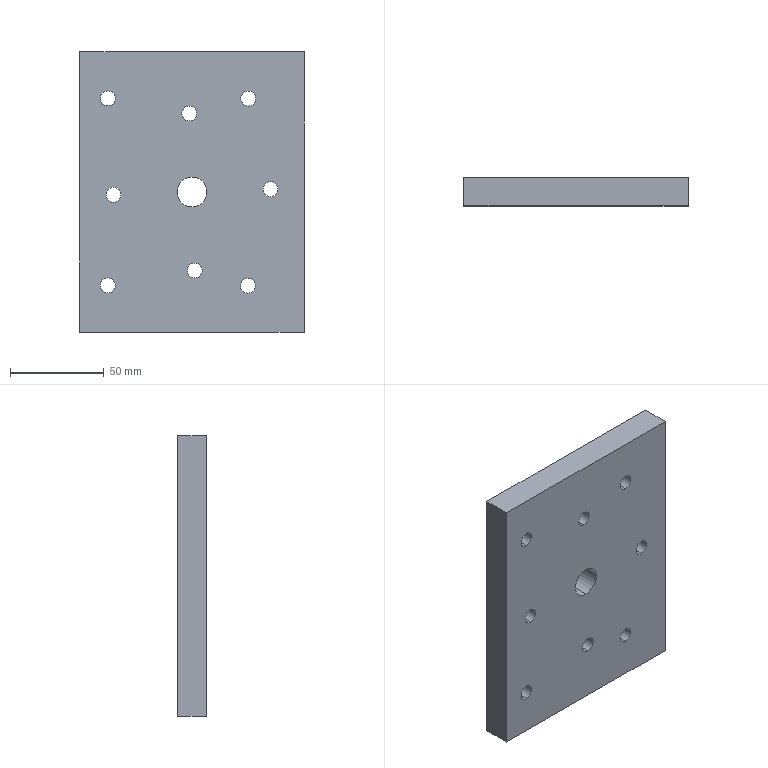Component | SolidWorks | ColumnSmallArmConnectionPlate-1 | 1 solid | 24 faces | box 120.16 x 15 x 150.13 mm | volume 260952 mm3 | cylinder 18 | plane 6 | commonest cylinder face diameters 8 x16 16 x2
build123d program:
from build123d import *

# Parameters (mm, degrees)
SKETCH1_W              = 120
SKETCH1_H              = 150
BOSS_EXTRUDE1_DEPTH    = 15
M8_TAPPED_HOLE2_D      = 8
M8_TAPPED_HOLE2_DEPTH  = 25
M8_TAPPED_HOLE2_TIP    = 2.403
M16_TAPPED_HOLE1_D     = 16
M16_TAPPED_HOLE1_DEPTH = 25
M16_TAPPED_HOLE1_TIP   = 4.807
M8_TAPPED_HOLE1_D      = 8
M8_TAPPED_HOLE1_DEPTH  = 25
M8_TAPPED_HOLE1_TIP    = 2.403


with BuildPart() as part:
    # Sketch1 → Boss-Extrude1 (new body)
    with BuildSketch(Plane(origin=(0, 0, 0), x_dir=(1, 0, 0), z_dir=(0, 1, 0))):
        Rectangle(SKETCH1_W, SKETCH1_H)
    extrude(amount=BOSS_EXTRUDE1_DEPTH)

    # M8 Tapped Hole2
    with Locations(Plane(origin=(0, 0, 0), x_dir=(-1, 0, 0), z_dir=(0, -1, 0))):
        with Locations((-41.973, -1.511), (1.511, -41.973), (41.973, 1.511), (-1.511, 41.973)):
            Hole(M8_TAPPED_HOLE2_D / 2, depth=M8_TAPPED_HOLE2_DEPTH)
            with Locations((0, 0, -(M8_TAPPED_HOLE2_DEPTH + M8_TAPPED_HOLE2_TIP / 2))):  # 118° drill point
                Cone(0, M8_TAPPED_HOLE2_D / 2, M8_TAPPED_HOLE2_TIP, mode=Mode.SUBTRACT)

    # M16 Tapped Hole1
    with Locations(Plane(origin=(0, 0, 0), x_dir=(-1, 0, 0), z_dir=(0, -1, 0))):
        with Locations((0, 0)):
            Hole(M16_TAPPED_HOLE1_D / 2, depth=M16_TAPPED_HOLE1_DEPTH)
            with Locations((0, 0, -(M16_TAPPED_HOLE1_DEPTH + M16_TAPPED_HOLE1_TIP / 2))):  # 118° drill point
                Cone(0, M16_TAPPED_HOLE1_D / 2, M16_TAPPED_HOLE1_TIP, mode=Mode.SUBTRACT)

    # M8 Tapped Hole1
    with Locations(Plane(origin=(0, 15, 0), x_dir=(1, 0, 0), z_dir=(0, 1, 0))):
        with Locations((-45, 50), (30, 50), (30, -50), (-45, -50)):
            Hole(M8_TAPPED_HOLE1_D / 2, depth=M8_TAPPED_HOLE1_DEPTH)
            with Locations((0, 0, -(M8_TAPPED_HOLE1_DEPTH + M8_TAPPED_HOLE1_TIP / 2))):  # 118° drill point
                Cone(0, M8_TAPPED_HOLE1_D / 2, M8_TAPPED_HOLE1_TIP, mode=Mode.SUBTRACT)


solid = part.part

# Placed as in the assembly
solid = solid.moved(Location((-87.309, 791.583, 566.392), (0, 0.0619, 0)))
STEP:
#1=COLOUR_RGB('',0.7922,0.8196,0.9333);
#2=FILL_AREA_STYLE_COLOUR('',#1);
#3=FILL_AREA_STYLE('',(#2));
#4=SURFACE_STYLE_FILL_AREA(#3);
#5=SURFACE_SIDE_STYLE('',(#4));
#6=SURFACE_STYLE_USAGE(.BOTH.,#5);
#7=PRESENTATION_STYLE_ASSIGNMENT((#6));
#8=CARTESIAN_POINT('',(-5.211,31.165,20.175));
#9=VERTEX_POINT('',#8);
#10=CARTESIAN_POINT('',(-5.211,31.165,20.49));
#11=VERTEX_POINT('',#10);
#12=CARTESIAN_POINT('',(-5.211,31.165,20.332));
#13=DIRECTION('',(0.,1.,-0.));
#14=DIRECTION('',(0.00108,0.,1.));
#15=AXIS2_PLACEMENT_3D('',#12,#13,#14);
#16=CIRCLE('',#15,0.1575);
#17=EDGE_CURVE('',#9,#11,#16,.T.);
#18=ORIENTED_EDGE('',*,*,#17,.F.);
#19=CARTESIAN_POINT('',(-5.211,31.755,20.175));
#20=VERTEX_POINT('',#19);
#21=CARTESIAN_POINT('',(-5.211,31.755,20.175));
#22=DIRECTION('',(0.,1.,-0.));
#23=VECTOR('',#22,39.37);
#24=LINE('',#21,#23);
#25=EDGE_CURVE('',#9,#20,#24,.T.);
#26=ORIENTED_EDGE('',*,*,#25,.T.);
#27=CARTESIAN_POINT('',(-5.211,31.755,20.49));
#28=VERTEX_POINT('',#27);
#29=CARTESIAN_POINT('',(-5.211,31.755,20.332));
#30=DIRECTION('',(0.,1.,-0.));
#31=DIRECTION('',(0.00108,0.,1.));
#32=AXIS2_PLACEMENT_3D('',#29,#30,#31);
#33=CIRCLE('',#32,0.1575);
#34=EDGE_CURVE('',#20,#28,#33,.T.);
#35=ORIENTED_EDGE('',*,*,#34,.T.);
#36=CARTESIAN_POINT('',(-5.211,31.755,20.49));
#37=DIRECTION('',(0.,1.,-0.));
#38=VECTOR('',#37,39.37);
#39=LINE('',#36,#38);
#40=EDGE_CURVE('',#11,#28,#39,.T.);
#41=ORIENTED_EDGE('',*,*,#40,.F.);
#42=EDGE_LOOP('',(#18,#26,#35,#41));
#43=FACE_OUTER_BOUND('',#42,.T.);
#44=CARTESIAN_POINT('',(-5.211,31.755,20.332));
#45=DIRECTION('',(0.,1.,-0.));
#46=DIRECTION('',(0.00108,0.,1.));
#47=AXIS2_PLACEMENT_3D('',#44,#45,#46);
#48=CYLINDRICAL_SURFACE('',#47,0.1575);
#49=ADVANCED_FACE('',(#43),#48,.F.);
#50=CARTESIAN_POINT('',(-2.259,31.165,20.172));
#51=VERTEX_POINT('',#50);
#52=CARTESIAN_POINT('',(-2.258,31.165,20.487));
#53=VERTEX_POINT('',#52);
#54=CARTESIAN_POINT('',(-2.258,31.165,20.329));
#55=DIRECTION('',(0.,1.,-0.));
#56=DIRECTION('',(0.00108,0.,1.));
#57=AXIS2_PLACEMENT_3D('',#54,#55,#56);
#58=CIRCLE('',#57,0.1575);
#59=EDGE_CURVE('',#51,#53,#58,.T.);
#60=ORIENTED_EDGE('',*,*,#59,.F.);
#61=CARTESIAN_POINT('',(-2.259,31.755,20.172));
#62=VERTEX_POINT('',#61);
#63=CARTESIAN_POINT('',(-2.259,31.755,20.172));
#64=DIRECTION('',(0.,1.,-0.));
#65=VECTOR('',#64,39.37);
#66=LINE('',#63,#65);
#67=EDGE_CURVE('',#51,#62,#66,.T.);
#68=ORIENTED_EDGE('',*,*,#67,.T.);
#69=CARTESIAN_POINT('',(-2.258,31.755,20.487));
#70=VERTEX_POINT('',#69);
#71=CARTESIAN_POINT('',(-2.258,31.755,20.329));
#72=DIRECTION('',(0.,1.,-0.));
#73=DIRECTION('',(0.00108,0.,1.));
#74=AXIS2_PLACEMENT_3D('',#71,#72,#73);
#75=CIRCLE('',#74,0.1575);
#76=EDGE_CURVE('',#62,#70,#75,.T.);
#77=ORIENTED_EDGE('',*,*,#76,.T.);
#78=CARTESIAN_POINT('',(-2.258,31.755,20.487));
#79=DIRECTION('',(0.,1.,-0.));
#80=VECTOR('',#79,39.37);
#81=LINE('',#78,#80);
#82=EDGE_CURVE('',#53,#70,#81,.T.);
#83=ORIENTED_EDGE('',*,*,#82,.F.);
#84=EDGE_LOOP('',(#60,#68,#77,#83));
#85=FACE_OUTER_BOUND('',#84,.T.);
#86=CARTESIAN_POINT('',(-2.258,31.755,20.329));
#87=DIRECTION('',(0.,1.,-0.));
#88=DIRECTION('',(0.00108,0.,1.));
#89=AXIS2_PLACEMENT_3D('',#86,#87,#88);
#90=CYLINDRICAL_SURFACE('',#89,0.1575);
#91=ADVANCED_FACE('',(#85),#90,.F.);
#92=CARTESIAN_POINT('',(-2.254,31.165,24.109));
#93=VERTEX_POINT('',#92);
#94=CARTESIAN_POINT('',(-2.254,31.165,24.424));
#95=VERTEX_POINT('',#94);
#96=CARTESIAN_POINT('',(-2.254,31.165,24.266));
#97=DIRECTION('',(0.,1.,-0.));
#98=DIRECTION('',(0.00108,0.,1.));
#99=AXIS2_PLACEMENT_3D('',#96,#97,#98);
#100=CIRCLE('',#99,0.1575);
#101=EDGE_CURVE('',#93,#95,#100,.T.);
#102=ORIENTED_EDGE('',*,*,#101,.F.);
#103=CARTESIAN_POINT('',(-2.254,31.755,24.109));
#104=VERTEX_POINT('',#103);
#105=CARTESIAN_POINT('',(-2.254,31.755,24.109));
#106=DIRECTION('',(0.,1.,-0.));
#107=VECTOR('',#106,39.37);
#108=LINE('',#105,#107);
#109=EDGE_CURVE('',#93,#104,#108,.T.);
#110=ORIENTED_EDGE('',*,*,#109,.T.);
#111=CARTESIAN_POINT('',(-2.254,31.755,24.424));
#112=VERTEX_POINT('',#111);
#113=CARTESIAN_POINT('',(-2.254,31.755,24.266));
#114=DIRECTION('',(0.,1.,-0.));
#115=DIRECTION('',(0.00108,0.,1.));
#116=AXIS2_PLACEMENT_3D('',#113,#114,#115);
#117=CIRCLE('',#116,0.1575);
#118=EDGE_CURVE('',#104,#112,#117,.T.);
#119=ORIENTED_EDGE('',*,*,#118,.T.);
#120=CARTESIAN_POINT('',(-2.254,31.755,24.424));
#121=DIRECTION('',(0.,1.,-0.));
#122=VECTOR('',#121,39.37);
#123=LINE('',#120,#122);
#124=EDGE_CURVE('',#95,#112,#123,.T.);
#125=ORIENTED_EDGE('',*,*,#124,.F.);
#126=EDGE_LOOP('',(#102,#110,#119,#125));
#127=FACE_OUTER_BOUND('',#126,.T.);
#128=CARTESIAN_POINT('',(-2.254,31.755,24.266));
#129=DIRECTION('',(0.,1.,-0.));
#130=DIRECTION('',(0.00108,0.,1.));
#131=AXIS2_PLACEMENT_3D('',#128,#129,#130);
#132=CYLINDRICAL_SURFACE('',#131,0.1575);
#133=ADVANCED_FACE('',(#127),#132,.F.);
#134=CARTESIAN_POINT('',(-5.207,31.165,24.112));
#135=VERTEX_POINT('',#134);
#136=CARTESIAN_POINT('',(-5.207,31.165,24.427));
#137=VERTEX_POINT('',#136);
#138=CARTESIAN_POINT('',(-5.207,31.165,24.269));
#139=DIRECTION('',(0.,1.,-0.));
#140=DIRECTION('',(0.00108,0.,1.));
#141=AXIS2_PLACEMENT_3D('',#138,#139,#140);
#142=CIRCLE('',#141,0.1575);
#143=EDGE_CURVE('',#135,#137,#142,.T.);
#144=ORIENTED_EDGE('',*,*,#143,.F.);
#145=CARTESIAN_POINT('',(-5.207,31.755,24.112));
#146=VERTEX_POINT('',#145);
#147=CARTESIAN_POINT('',(-5.207,31.755,24.112));
#148=DIRECTION('',(0.,1.,-0.));
#149=VECTOR('',#148,39.37);
#150=LINE('',#147,#149);
#151=EDGE_CURVE('',#135,#146,#150,.T.);
#152=ORIENTED_EDGE('',*,*,#151,.T.);
#153=CARTESIAN_POINT('',(-5.207,31.755,24.427));
#154=VERTEX_POINT('',#153);
#155=CARTESIAN_POINT('',(-5.207,31.755,24.269));
#156=DIRECTION('',(0.,1.,-0.));
#157=DIRECTION('',(0.00108,0.,1.));
#158=AXIS2_PLACEMENT_3D('',#155,#156,#157);
#159=CIRCLE('',#158,0.1575);
#160=EDGE_CURVE('',#146,#154,#159,.T.);
#161=ORIENTED_EDGE('',*,*,#160,.T.);
#162=CARTESIAN_POINT('',(-5.207,31.755,24.427));
#163=DIRECTION('',(0.,1.,-0.));
#164=VECTOR('',#163,39.37);
#165=LINE('',#162,#164);
#166=EDGE_CURVE('',#137,#154,#165,.T.);
#167=ORIENTED_EDGE('',*,*,#166,.F.);
#168=EDGE_LOOP('',(#144,#152,#161,#167));
#169=FACE_OUTER_BOUND('',#168,.T.);
#170=CARTESIAN_POINT('',(-5.207,31.755,24.269));
#171=DIRECTION('',(0.,1.,-0.));
#172=DIRECTION('',(0.00108,0.,1.));
#173=AXIS2_PLACEMENT_3D('',#170,#171,#172);
#174=CYLINDRICAL_SURFACE('',#173,0.1575);
#175=ADVANCED_FACE('',(#169),#174,.F.);
#176=CARTESIAN_POINT('',(-3.438,31.755,21.984));
#177=VERTEX_POINT('',#176);
#178=CARTESIAN_POINT('',(-3.437,31.755,22.614));
#179=VERTEX_POINT('',#178);
#180=CARTESIAN_POINT('',(-3.437,31.755,22.299));
#181=DIRECTION('',(0.,1.,-0.));
#182=DIRECTION('',(0.00108,0.,1.));
#183=AXIS2_PLACEMENT_3D('',#180,#181,#182);
#184=CIRCLE('',#183,0.315);
#185=EDGE_CURVE('',#177,#179,#184,.T.);
#186=ORIENTED_EDGE('',*,*,#185,.T.);
#187=CARTESIAN_POINT('',(-3.437,31.165,22.614));
#188=VERTEX_POINT('',#187);
#189=CARTESIAN_POINT('',(-3.437,31.165,22.614));
#190=DIRECTION('',(-0.,-1.,0.));
#191=VECTOR('',#190,39.37);
#192=LINE('',#189,#191);
#193=EDGE_CURVE('',#179,#188,#192,.T.);
#194=ORIENTED_EDGE('',*,*,#193,.T.);
#195=CARTESIAN_POINT('',(-3.438,31.165,21.984));
#196=VERTEX_POINT('',#195);
#197=CARTESIAN_POINT('',(-3.437,31.165,22.299));
#198=DIRECTION('',(-0.,-1.,0.));
#199=DIRECTION('',(-0.00108,0.,-1.));
#200=AXIS2_PLACEMENT_3D('',#197,#198,#199);
#201=CIRCLE('',#200,0.315);
#202=EDGE_CURVE('',#188,#196,#201,.T.);
#203=ORIENTED_EDGE('',*,*,#202,.T.);
#204=CARTESIAN_POINT('',(-3.438,31.165,21.984));
#205=DIRECTION('',(-0.,-1.,0.));
#206=VECTOR('',#205,39.37);
#207=LINE('',#204,#206);
#208=EDGE_CURVE('',#177,#196,#207,.T.);
#209=ORIENTED_EDGE('',*,*,#208,.F.);
#210=EDGE_LOOP('',(#186,#194,#203,#209));
#211=FACE_OUTER_BOUND('',#210,.T.);
#212=CARTESIAN_POINT('',(-3.437,31.165,22.299));
#213=DIRECTION('',(-0.,-1.,0.));
#214=DIRECTION('',(-0.00108,0.,-1.));
#215=AXIS2_PLACEMENT_3D('',#212,#213,#214);
#216=CYLINDRICAL_SURFACE('',#215,0.315);
#217=ADVANCED_FACE('',(#211),#216,.F.);
#218=CARTESIAN_POINT('',(-1.785,31.755,22.199));
#219=VERTEX_POINT('',#218);
#220=CARTESIAN_POINT('',(-1.785,31.755,22.514));
#221=VERTEX_POINT('',#220);
#222=CARTESIAN_POINT('',(-1.785,31.755,22.357));
#223=DIRECTION('',(0.,1.,-0.));
#224=DIRECTION('',(0.00108,0.,1.));
#225=AXIS2_PLACEMENT_3D('',#222,#223,#224);
#226=CIRCLE('',#225,0.1575);
#227=EDGE_CURVE('',#219,#221,#226,.T.);
#228=ORIENTED_EDGE('',*,*,#227,.T.);
#229=CARTESIAN_POINT('',(-1.785,31.165,22.514));
#230=VERTEX_POINT('',#229);
#231=CARTESIAN_POINT('',(-1.785,31.165,22.514));
#232=DIRECTION('',(-0.,-1.,0.));
#233=VECTOR('',#232,39.37);
#234=LINE('',#231,#233);
#235=EDGE_CURVE('',#221,#230,#234,.T.);
#236=ORIENTED_EDGE('',*,*,#235,.T.);
#237=CARTESIAN_POINT('',(-1.785,31.165,22.199));
#238=VERTEX_POINT('',#237);
#239=CARTESIAN_POINT('',(-1.785,31.165,22.357));
#240=DIRECTION('',(-0.,-1.,0.));
#241=DIRECTION('',(-0.00108,0.,-1.));
#242=AXIS2_PLACEMENT_3D('',#239,#240,#241);
#243=CIRCLE('',#242,0.1575);
#244=EDGE_CURVE('',#230,#238,#243,.T.);
#245=ORIENTED_EDGE('',*,*,#244,.T.);
#246=CARTESIAN_POINT('',(-1.785,31.165,22.199));
#247=DIRECTION('',(-0.,-1.,0.));
#248=VECTOR('',#247,39.37);
#249=LINE('',#246,#248);
#250=EDGE_CURVE('',#219,#238,#249,.T.);
#251=ORIENTED_EDGE('',*,*,#250,.F.);
#252=EDGE_LOOP('',(#228,#236,#245,#251));
#253=FACE_OUTER_BOUND('',#252,.T.);
#254=CARTESIAN_POINT('',(-1.785,31.165,22.357));
#255=DIRECTION('',(-0.,-1.,0.));
#256=DIRECTION('',(-0.00108,0.,-1.));
#257=AXIS2_PLACEMENT_3D('',#254,#255,#256);
#258=CYLINDRICAL_SURFACE('',#257,0.1575);
#259=ADVANCED_FACE('',(#253),#258,.F.);
#260=CARTESIAN_POINT('',(-3.495,31.755,23.794));
#261=VERTEX_POINT('',#260);
#262=CARTESIAN_POINT('',(-3.495,31.755,24.109));
#263=VERTEX_POINT('',#262);
#264=CARTESIAN_POINT('',(-3.495,31.755,23.951));
#265=DIRECTION('',(0.,1.,-0.));
#266=DIRECTION('',(0.00108,0.,1.));
#267=AXIS2_PLACEMENT_3D('',#264,#265,#266);
#268=CIRCLE('',#267,0.1575);
#269=EDGE_CURVE('',#261,#263,#268,.T.);
#270=ORIENTED_EDGE('',*,*,#269,.T.);
#271=CARTESIAN_POINT('',(-3.495,31.165,24.109));
#272=VERTEX_POINT('',#271);
#273=CARTESIAN_POINT('',(-3.495,31.165,24.109));
#274=DIRECTION('',(-0.,-1.,0.));
#275=VECTOR('',#274,39.37);
#276=LINE('',#273,#275);
#277=EDGE_CURVE('',#263,#272,#276,.T.);
#278=ORIENTED_EDGE('',*,*,#277,.T.);
#279=CARTESIAN_POINT('',(-3.495,31.165,23.794));
#280=VERTEX_POINT('',#279);
#281=CARTESIAN_POINT('',(-3.495,31.165,23.951));
#282=DIRECTION('',(-0.,-1.,0.));
#283=DIRECTION('',(-0.00108,0.,-1.));
#284=AXIS2_PLACEMENT_3D('',#281,#282,#283);
#285=CIRCLE('',#284,0.1575);
#286=EDGE_CURVE('',#272,#280,#285,.T.);
#287=ORIENTED_EDGE('',*,*,#286,.T.);
#288=CARTESIAN_POINT('',(-3.495,31.165,23.794));
#289=DIRECTION('',(-0.,-1.,0.));
#290=VECTOR('',#289,39.37);
#291=LINE('',#288,#290);
#292=EDGE_CURVE('',#261,#280,#291,.T.);
#293=ORIENTED_EDGE('',*,*,#292,.F.);
#294=EDGE_LOOP('',(#270,#278,#287,#293));
#295=FACE_OUTER_BOUND('',#294,.T.);
#296=CARTESIAN_POINT('',(-3.495,31.165,23.951));
#297=DIRECTION('',(-0.,-1.,0.));
#298=DIRECTION('',(-0.00108,0.,-1.));
#299=AXIS2_PLACEMENT_3D('',#296,#297,#298);
#300=CYLINDRICAL_SURFACE('',#299,0.1575);
#301=ADVANCED_FACE('',(#295),#300,.F.);
#302=CARTESIAN_POINT('',(-5.09,31.755,22.084));
#303=VERTEX_POINT('',#302);
#304=CARTESIAN_POINT('',(-5.09,31.755,22.399));
#305=VERTEX_POINT('',#304);
#306=CARTESIAN_POINT('',(-5.09,31.755,22.241));
#307=DIRECTION('',(0.,1.,-0.));
#308=DIRECTION('',(0.00108,0.,1.));
#309=AXIS2_PLACEMENT_3D('',#306,#307,#308);
#310=CIRCLE('',#309,0.1575);
#311=EDGE_CURVE('',#303,#305,#310,.T.);
#312=ORIENTED_EDGE('',*,*,#311,.T.);
#313=CARTESIAN_POINT('',(-5.09,31.165,22.399));
#314=VERTEX_POINT('',#313);
#315=CARTESIAN_POINT('',(-5.09,31.165,22.399));
#316=DIRECTION('',(-0.,-1.,0.));
#317=VECTOR('',#316,39.37);
#318=LINE('',#315,#317);
#319=EDGE_CURVE('',#305,#314,#318,.T.);
#320=ORIENTED_EDGE('',*,*,#319,.T.);
#321=CARTESIAN_POINT('',(-5.09,31.165,22.084));
#322=VERTEX_POINT('',#321);
#323=CARTESIAN_POINT('',(-5.09,31.165,22.241));
#324=DIRECTION('',(-0.,-1.,0.));
#325=DIRECTION('',(-0.00108,0.,-1.));
#326=AXIS2_PLACEMENT_3D('',#323,#324,#325);
#327=CIRCLE('',#326,0.1575);
#328=EDGE_CURVE('',#314,#322,#327,.T.);
#329=ORIENTED_EDGE('',*,*,#328,.T.);
#330=CARTESIAN_POINT('',(-5.09,31.165,22.084));
#331=DIRECTION('',(-0.,-1.,0.));
#332=VECTOR('',#331,39.37);
#333=LINE('',#330,#332);
#334=EDGE_CURVE('',#303,#322,#333,.T.);
#335=ORIENTED_EDGE('',*,*,#334,.F.);
#336=EDGE_LOOP('',(#312,#320,#329,#335));
#337=FACE_OUTER_BOUND('',#336,.T.);
#338=CARTESIAN_POINT('',(-5.09,31.165,22.241));
#339=DIRECTION('',(-0.,-1.,0.));
#340=DIRECTION('',(-0.00108,0.,-1.));
#341=AXIS2_PLACEMENT_3D('',#338,#339,#340);
#342=CYLINDRICAL_SURFACE('',#341,0.1575);
#343=ADVANCED_FACE('',(#337),#342,.F.);
#344=CARTESIAN_POINT('',(-3.38,31.755,20.489));
#345=VERTEX_POINT('',#344);
#346=CARTESIAN_POINT('',(-3.379,31.755,20.804));
#347=VERTEX_POINT('',#346);
#348=CARTESIAN_POINT('',(-3.38,31.755,20.646));
#349=DIRECTION('',(0.,1.,-0.));
#350=DIRECTION('',(0.00108,0.,1.));
#351=AXIS2_PLACEMENT_3D('',#348,#349,#350);
#352=CIRCLE('',#351,0.1575);
#353=EDGE_CURVE('',#345,#347,#352,.T.);
#354=ORIENTED_EDGE('',*,*,#353,.T.);
#355=CARTESIAN_POINT('',(-3.379,31.165,20.804));
#356=VERTEX_POINT('',#355);
#357=CARTESIAN_POINT('',(-3.379,31.165,20.804));
#358=DIRECTION('',(-0.,-1.,0.));
#359=VECTOR('',#358,39.37);
#360=LINE('',#357,#359);
#361=EDGE_CURVE('',#347,#356,#360,.T.);
#362=ORIENTED_EDGE('',*,*,#361,.T.);
#363=CARTESIAN_POINT('',(-3.38,31.165,20.489));
#364=VERTEX_POINT('',#363);
#365=CARTESIAN_POINT('',(-3.38,31.165,20.646));
#366=DIRECTION('',(-0.,-1.,0.));
#367=DIRECTION('',(-0.00108,0.,-1.));
#368=AXIS2_PLACEMENT_3D('',#365,#366,#367);
#369=CIRCLE('',#368,0.1575);
#370=EDGE_CURVE('',#356,#364,#369,.T.);
#371=ORIENTED_EDGE('',*,*,#370,.T.);
#372=CARTESIAN_POINT('',(-3.38,31.165,20.489));
#373=DIRECTION('',(-0.,-1.,0.));
#374=VECTOR('',#373,39.37);
#375=LINE('',#372,#374);
#376=EDGE_CURVE('',#345,#364,#375,.T.);
#377=ORIENTED_EDGE('',*,*,#376,.F.);
#378=EDGE_LOOP('',(#354,#362,#371,#377));
#379=FACE_OUTER_BOUND('',#378,.T.);
#380=CARTESIAN_POINT('',(-3.38,31.165,20.646));
#381=DIRECTION('',(-0.,-1.,0.));
#382=DIRECTION('',(-0.00108,0.,-1.));
#383=AXIS2_PLACEMENT_3D('',#380,#381,#382);
#384=CYLINDRICAL_SURFACE('',#383,0.1575);
#385=ADVANCED_FACE('',(#379),#384,.F.);
#386=CARTESIAN_POINT('',(-5.803,31.165,19.349));
#387=VERTEX_POINT('',#386);
#388=CARTESIAN_POINT('',(-5.796,31.165,25.254));
#389=VERTEX_POINT('',#388);
#390=CARTESIAN_POINT('',(-5.796,31.165,25.254));
#391=DIRECTION('',(0.00108,0.,1.));
#392=VECTOR('',#391,39.37);
#393=LINE('',#390,#392);
#394=EDGE_CURVE('',#387,#389,#393,.T.);
#395=ORIENTED_EDGE('',*,*,#394,.T.);
#396=CARTESIAN_POINT('',(-5.796,31.755,25.254));
#397=VERTEX_POINT('',#396);
#398=CARTESIAN_POINT('',(-5.796,31.755,25.254));
#399=DIRECTION('',(-0.,-1.,0.));
#400=VECTOR('',#399,39.37);
#401=LINE('',#398,#400);
#402=EDGE_CURVE('',#397,#389,#401,.T.);
#403=ORIENTED_EDGE('',*,*,#402,.F.);
#404=CARTESIAN_POINT('',(-5.803,31.755,19.349));
#405=VERTEX_POINT('',#404);
#406=CARTESIAN_POINT('',(-5.796,31.755,25.254));
#407=DIRECTION('',(0.00108,0.,1.));
#408=VECTOR('',#407,39.37);
#409=LINE('',#406,#408);
#410=EDGE_CURVE('',#405,#397,#409,.T.);
#411=ORIENTED_EDGE('',*,*,#410,.F.);
#412=CARTESIAN_POINT('',(-5.803,31.755,19.349));
#413=DIRECTION('',(-0.,-1.,0.));
#414=VECTOR('',#413,39.37);
#415=LINE('',#412,#414);
#416=EDGE_CURVE('',#405,#387,#415,.T.);
#417=ORIENTED_EDGE('',*,*,#416,.T.);
#418=EDGE_LOOP('',(#395,#403,#411,#417));
#419=FACE_OUTER_BOUND('',#418,.T.);
#420=CARTESIAN_POINT('',(-5.796,31.755,25.254));
#421=DIRECTION('',(1.,-0.,-0.00108));
#422=DIRECTION('',(-0.00108,-0.,-1.));
#423=AXIS2_PLACEMENT_3D('',#420,#421,#422);
#424=PLANE('',#423);
#425=ADVANCED_FACE('',(#419),#424,.F.);
#426=CARTESIAN_POINT('',(-1.072,31.165,25.249));
#427=VERTEX_POINT('',#426);
#428=CARTESIAN_POINT('',(-1.072,31.165,25.249));
#429=DIRECTION('',(1.,-0.,-0.00108));
#430=VECTOR('',#429,39.37);
#431=LINE('',#428,#430);
#432=EDGE_CURVE('',#389,#427,#431,.T.);
#433=ORIENTED_EDGE('',*,*,#432,.T.);
#434=CARTESIAN_POINT('',(-1.072,31.755,25.249));
#435=VERTEX_POINT('',#434);
#436=CARTESIAN_POINT('',(-1.072,31.755,25.249));
#437=DIRECTION('',(-0.,-1.,0.));
#438=VECTOR('',#437,39.37);
#439=LINE('',#436,#438);
#440=EDGE_CURVE('',#435,#427,#439,.T.);
#441=ORIENTED_EDGE('',*,*,#440,.F.);
#442=CARTESIAN_POINT('',(-1.072,31.755,25.249));
#443=DIRECTION('',(1.,-0.,-0.00108));
#444=VECTOR('',#443,39.37);
#445=LINE('',#442,#444);
#446=EDGE_CURVE('',#397,#435,#445,.T.);
#447=ORIENTED_EDGE('',*,*,#446,.F.);
#448=ORIENTED_EDGE('',*,*,#402,.T.);
#449=EDGE_LOOP('',(#433,#441,#447,#448));
#450=FACE_OUTER_BOUND('',#449,.T.);
#451=CARTESIAN_POINT('',(-1.072,31.755,25.249));
#452=DIRECTION('',(-0.00108,-0.,-1.));
#453=DIRECTION('',(-1.,0.,0.00108));
#454=AXIS2_PLACEMENT_3D('',#451,#452,#453);
#455=PLANE('',#454);
#456=ADVANCED_FACE('',(#450),#455,.F.);
#457=CARTESIAN_POINT('',(-1.078,31.165,19.344));
#458=VERTEX_POINT('',#457);
#459=CARTESIAN_POINT('',(-1.072,31.165,25.249));
#460=DIRECTION('',(-0.00108,-0.,-1.));
#461=VECTOR('',#460,39.37);
#462=LINE('',#459,#461);
#463=EDGE_CURVE('',#427,#458,#462,.T.);
#464=ORIENTED_EDGE('',*,*,#463,.T.);
#465=CARTESIAN_POINT('',(-1.078,31.755,19.344));
#466=VERTEX_POINT('',#465);
#467=CARTESIAN_POINT('',(-1.078,31.755,19.344));
#468=DIRECTION('',(-0.,-1.,0.));
#469=VECTOR('',#468,39.37);
#470=LINE('',#467,#469);
#471=EDGE_CURVE('',#466,#458,#470,.T.);
#472=ORIENTED_EDGE('',*,*,#471,.F.);
#473=CARTESIAN_POINT('',(-1.072,31.755,25.249));
#474=DIRECTION('',(-0.00108,-0.,-1.));
#475=VECTOR('',#474,39.37);
#476=LINE('',#473,#475);
#477=EDGE_CURVE('',#435,#466,#476,.T.);
#478=ORIENTED_EDGE('',*,*,#477,.F.);
#479=ORIENTED_EDGE('',*,*,#440,.T.);
#480=EDGE_LOOP('',(#464,#472,#478,#479));
#481=FACE_OUTER_BOUND('',#480,.T.);
#482=CARTESIAN_POINT('',(-1.072,31.755,25.249));
#483=DIRECTION('',(-1.,0.,0.00108));
#484=DIRECTION('',(0.00108,0.,1.));
#485=AXIS2_PLACEMENT_3D('',#482,#483,#484);
#486=PLANE('',#485);
#487=ADVANCED_FACE('',(#481),#486,.F.);
#488=CARTESIAN_POINT('',(-1.078,31.165,19.344));
#489=DIRECTION('',(-1.,0.,0.00108));
#490=VECTOR('',#489,39.37);
#491=LINE('',#488,#490);
#492=EDGE_CURVE('',#458,#387,#491,.T.);
#493=ORIENTED_EDGE('',*,*,#492,.T.);
#494=ORIENTED_EDGE('',*,*,#416,.F.);
#495=CARTESIAN_POINT('',(-1.078,31.755,19.344));
#496=DIRECTION('',(-1.,0.,0.00108));
#497=VECTOR('',#496,39.37);
#498=LINE('',#495,#497);
#499=EDGE_CURVE('',#466,#405,#498,.T.);
#500=ORIENTED_EDGE('',*,*,#499,.F.);
#501=ORIENTED_EDGE('',*,*,#471,.T.);
#502=EDGE_LOOP('',(#493,#494,#500,#501));
#503=FACE_OUTER_BOUND('',#502,.T.);
#504=CARTESIAN_POINT('',(-1.078,31.755,19.344));
#505=DIRECTION('',(0.00108,0.,1.));
#506=DIRECTION('',(1.,-0.,-0.00108));
#507=AXIS2_PLACEMENT_3D('',#504,#505,#506);
#508=PLANE('',#507);
#509=ADVANCED_FACE('',(#503),#508,.F.);
#510=CARTESIAN_POINT('',(-5.211,31.755,20.332));
#511=DIRECTION('',(0.,1.,-0.));
#512=DIRECTION('',(0.00108,0.,1.));
#513=AXIS2_PLACEMENT_3D('',#510,#511,#512);
#514=CIRCLE('',#513,0.1575);
#515=EDGE_CURVE('',#28,#20,#514,.T.);
#516=ORIENTED_EDGE('',*,*,#515,.F.);
#517=ORIENTED_EDGE('',*,*,#34,.F.);
#518=EDGE_LOOP('',(#516,#517));
#519=FACE_BOUND('',#518,.T.);
#520=CARTESIAN_POINT('',(-2.258,31.755,20.329));
#521=DIRECTION('',(0.,1.,-0.));
#522=DIRECTION('',(0.00108,0.,1.));
#523=AXIS2_PLACEMENT_3D('',#520,#521,#522);
#524=CIRCLE('',#523,0.1575);
#525=EDGE_CURVE('',#70,#62,#524,.T.);
#526=ORIENTED_EDGE('',*,*,#525,.F.);
#527=ORIENTED_EDGE('',*,*,#76,.F.);
#528=EDGE_LOOP('',(#526,#527));
#529=FACE_BOUND('',#528,.T.);
#530=CARTESIAN_POINT('',(-2.254,31.755,24.266));
#531=DIRECTION('',(0.,1.,-0.));
#532=DIRECTION('',(0.00108,0.,1.));
#533=AXIS2_PLACEMENT_3D('',#530,#531,#532);
#534=CIRCLE('',#533,0.1575);
#535=EDGE_CURVE('',#112,#104,#534,.T.);
#536=ORIENTED_EDGE('',*,*,#535,.F.);
#537=ORIENTED_EDGE('',*,*,#118,.F.);
#538=EDGE_LOOP('',(#536,#537));
#539=FACE_BOUND('',#538,.T.);
#540=CARTESIAN_POINT('',(-5.207,31.755,24.269));
#541=DIRECTION('',(0.,1.,-0.));
#542=DIRECTION('',(0.00108,0.,1.));
#543=AXIS2_PLACEMENT_3D('',#540,#541,#542);
#544=CIRCLE('',#543,0.1575);
#545=EDGE_CURVE('',#154,#146,#544,.T.);
#546=ORIENTED_EDGE('',*,*,#545,.F.);
#547=ORIENTED_EDGE('',*,*,#160,.F.);
#548=EDGE_LOOP('',(#546,#547));
#549=FACE_BOUND('',#548,.T.);
#550=ORIENTED_EDGE('',*,*,#185,.F.);
#551=CARTESIAN_POINT('',(-3.437,31.755,22.299));
#552=DIRECTION('',(0.,1.,-0.));
#553=DIRECTION('',(0.00108,0.,1.));
#554=AXIS2_PLACEMENT_3D('',#551,#552,#553);
#555=CIRCLE('',#554,0.315);
#556=EDGE_CURVE('',#179,#177,#555,.T.);
#557=ORIENTED_EDGE('',*,*,#556,.F.);
#558=EDGE_LOOP('',(#550,#557));
#559=FACE_BOUND('',#558,.T.);
#560=ORIENTED_EDGE('',*,*,#227,.F.);
#561=CARTESIAN_POINT('',(-1.785,31.755,22.357));
#562=DIRECTION('',(0.,1.,-0.));
#563=DIRECTION('',(0.00108,0.,1.));
#564=AXIS2_PLACEMENT_3D('',#561,#562,#563);
#565=CIRCLE('',#564,0.1575);
#566=EDGE_CURVE('',#221,#219,#565,.T.);
#567=ORIENTED_EDGE('',*,*,#566,.F.);
#568=EDGE_LOOP('',(#560,#567));
#569=FACE_BOUND('',#568,.T.);
#570=ORIENTED_EDGE('',*,*,#269,.F.);
#571=CARTESIAN_POINT('',(-3.495,31.755,23.951));
#572=DIRECTION('',(0.,1.,-0.));
#573=DIRECTION('',(0.00108,0.,1.));
#574=AXIS2_PLACEMENT_3D('',#571,#572,#573);
#575=CIRCLE('',#574,0.1575);
#576=EDGE_CURVE('',#263,#261,#575,.T.);
#577=ORIENTED_EDGE('',*,*,#576,.F.);
#578=EDGE_LOOP('',(#570,#577));
#579=FACE_BOUND('',#578,.T.);
#580=ORIENTED_EDGE('',*,*,#311,.F.);
#581=CARTESIAN_POINT('',(-5.09,31.755,22.241));
#582=DIRECTION('',(0.,1.,-0.));
#583=DIRECTION('',(0.00108,0.,1.));
#584=AXIS2_PLACEMENT_3D('',#581,#582,#583);
#585=CIRCLE('',#584,0.1575);
#586=EDGE_CURVE('',#305,#303,#585,.T.);
#587=ORIENTED_EDGE('',*,*,#586,.F.);
#588=EDGE_LOOP('',(#580,#587));
#589=FACE_BOUND('',#588,.T.);
#590=ORIENTED_EDGE('',*,*,#353,.F.);
#591=CARTESIAN_POINT('',(-3.38,31.755,20.646));
#592=DIRECTION('',(0.,1.,-0.));
#593=DIRECTION('',(0.00108,0.,1.));
#594=AXIS2_PLACEMENT_3D('',#591,#592,#593);
#595=CIRCLE('',#594,0.1575);
#596=EDGE_CURVE('',#347,#345,#595,.T.);
#597=ORIENTED_EDGE('',*,*,#596,.F.);
#598=EDGE_LOOP('',(#590,#597));
#599=FACE_BOUND('',#598,.T.);
#600=ORIENTED_EDGE('',*,*,#410,.T.);
#601=ORIENTED_EDGE('',*,*,#446,.T.);
#602=ORIENTED_EDGE('',*,*,#477,.T.);
#603=ORIENTED_EDGE('',*,*,#499,.T.);
#604=EDGE_LOOP('',(#600,#601,#602,#603));
#605=FACE_OUTER_BOUND('',#604,.T.);
#606=CARTESIAN_POINT('',(-3.437,31.755,22.299));
#607=DIRECTION('',(0.,1.,-0.));
#608=DIRECTION('',(0.00108,0.,1.));
#609=AXIS2_PLACEMENT_3D('',#606,#607,#608);
#610=PLANE('',#609);
#611=ADVANCED_FACE('',(#519,#529,#539,#549,#559,#569,#579,#589,#599,#605),#610,.T.);
#612=CARTESIAN_POINT('',(-5.211,31.165,20.332));
#613=DIRECTION('',(0.,1.,-0.));
#614=DIRECTION('',(0.00108,0.,1.));
#615=AXIS2_PLACEMENT_3D('',#612,#613,#614);
#616=CIRCLE('',#615,0.1575);
#617=EDGE_CURVE('',#11,#9,#616,.T.);
#618=ORIENTED_EDGE('',*,*,#617,.T.);
#619=ORIENTED_EDGE('',*,*,#17,.T.);
#620=EDGE_LOOP('',(#618,#619));
#621=FACE_BOUND('',#620,.T.);
#622=CARTESIAN_POINT('',(-2.258,31.165,20.329));
#623=DIRECTION('',(0.,1.,-0.));
#624=DIRECTION('',(0.00108,0.,1.));
#625=AXIS2_PLACEMENT_3D('',#622,#623,#624);
#626=CIRCLE('',#625,0.1575);
#627=EDGE_CURVE('',#53,#51,#626,.T.);
#628=ORIENTED_EDGE('',*,*,#627,.T.);
#629=ORIENTED_EDGE('',*,*,#59,.T.);
#630=EDGE_LOOP('',(#628,#629));
#631=FACE_BOUND('',#630,.T.);
#632=CARTESIAN_POINT('',(-2.254,31.165,24.266));
#633=DIRECTION('',(0.,1.,-0.));
#634=DIRECTION('',(0.00108,0.,1.));
#635=AXIS2_PLACEMENT_3D('',#632,#633,#634);
#636=CIRCLE('',#635,0.1575);
#637=EDGE_CURVE('',#95,#93,#636,.T.);
#638=ORIENTED_EDGE('',*,*,#637,.T.);
#639=ORIENTED_EDGE('',*,*,#101,.T.);
#640=EDGE_LOOP('',(#638,#639));
#641=FACE_BOUND('',#640,.T.);
#642=CARTESIAN_POINT('',(-5.207,31.165,24.269));
#643=DIRECTION('',(0.,1.,-0.));
#644=DIRECTION('',(0.00108,0.,1.));
#645=AXIS2_PLACEMENT_3D('',#642,#643,#644);
#646=CIRCLE('',#645,0.1575);
#647=EDGE_CURVE('',#137,#135,#646,.T.);
#648=ORIENTED_EDGE('',*,*,#647,.T.);
#649=ORIENTED_EDGE('',*,*,#143,.T.);
#650=EDGE_LOOP('',(#648,#649));
#651=FACE_BOUND('',#650,.T.);
#652=CARTESIAN_POINT('',(-3.437,31.165,22.299));
#653=DIRECTION('',(-0.,-1.,0.));
#654=DIRECTION('',(-0.00108,0.,-1.));
#655=AXIS2_PLACEMENT_3D('',#652,#653,#654);
#656=CIRCLE('',#655,0.315);
#657=EDGE_CURVE('',#196,#188,#656,.T.);
#658=ORIENTED_EDGE('',*,*,#657,.F.);
#659=ORIENTED_EDGE('',*,*,#202,.F.);
#660=EDGE_LOOP('',(#658,#659));
#661=FACE_BOUND('',#660,.T.);
#662=CARTESIAN_POINT('',(-1.785,31.165,22.357));
#663=DIRECTION('',(-0.,-1.,0.));
#664=DIRECTION('',(-0.00108,0.,-1.));
#665=AXIS2_PLACEMENT_3D('',#662,#663,#664);
#666=CIRCLE('',#665,0.1575);
#667=EDGE_CURVE('',#238,#230,#666,.T.);
#668=ORIENTED_EDGE('',*,*,#667,.F.);
#669=ORIENTED_EDGE('',*,*,#244,.F.);
#670=EDGE_LOOP('',(#668,#669));
#671=FACE_BOUND('',#670,.T.);
#672=CARTESIAN_POINT('',(-3.495,31.165,23.951));
#673=DIRECTION('',(-0.,-1.,0.));
#674=DIRECTION('',(-0.00108,0.,-1.));
#675=AXIS2_PLACEMENT_3D('',#672,#673,#674);
#676=CIRCLE('',#675,0.1575);
#677=EDGE_CURVE('',#280,#272,#676,.T.);
#678=ORIENTED_EDGE('',*,*,#677,.F.);
#679=ORIENTED_EDGE('',*,*,#286,.F.);
#680=EDGE_LOOP('',(#678,#679));
#681=FACE_BOUND('',#680,.T.);
#682=CARTESIAN_POINT('',(-5.09,31.165,22.241));
#683=DIRECTION('',(-0.,-1.,0.));
#684=DIRECTION('',(-0.00108,0.,-1.));
#685=AXIS2_PLACEMENT_3D('',#682,#683,#684);
#686=CIRCLE('',#685,0.1575);
#687=EDGE_CURVE('',#322,#314,#686,.T.);
#688=ORIENTED_EDGE('',*,*,#687,.F.);
#689=ORIENTED_EDGE('',*,*,#328,.F.);
#690=EDGE_LOOP('',(#688,#689));
#691=FACE_BOUND('',#690,.T.);
#692=CARTESIAN_POINT('',(-3.38,31.165,20.646));
#693=DIRECTION('',(-0.,-1.,0.));
#694=DIRECTION('',(-0.00108,0.,-1.));
#695=AXIS2_PLACEMENT_3D('',#692,#693,#694);
#696=CIRCLE('',#695,0.1575);
#697=EDGE_CURVE('',#364,#356,#696,.T.);
#698=ORIENTED_EDGE('',*,*,#697,.F.);
#699=ORIENTED_EDGE('',*,*,#370,.F.);
#700=EDGE_LOOP('',(#698,#699));
#701=FACE_BOUND('',#700,.T.);
#702=ORIENTED_EDGE('',*,*,#394,.F.);
#703=ORIENTED_EDGE('',*,*,#492,.F.);
#704=ORIENTED_EDGE('',*,*,#463,.F.);
#705=ORIENTED_EDGE('',*,*,#432,.F.);
#706=EDGE_LOOP('',(#702,#703,#704,#705));
#707=FACE_OUTER_BOUND('',#706,.T.);
#708=CARTESIAN_POINT('',(-3.437,31.165,22.299));
#709=DIRECTION('',(0.,1.,-0.));
#710=DIRECTION('',(0.00108,0.,1.));
#711=AXIS2_PLACEMENT_3D('',#708,#709,#710);
#712=PLANE('',#711);
#713=ADVANCED_FACE('',(#621,#631,#641,#651,#661,#671,#681,#691,#701,#707),#712,.F.);
#714=ORIENTED_EDGE('',*,*,#361,.F.);
#715=ORIENTED_EDGE('',*,*,#596,.T.);
#716=ORIENTED_EDGE('',*,*,#376,.T.);
#717=ORIENTED_EDGE('',*,*,#697,.T.);
#718=EDGE_LOOP('',(#714,#715,#716,#717));
#719=FACE_OUTER_BOUND('',#718,.T.);
#720=CARTESIAN_POINT('',(-3.38,31.165,20.646));
#721=DIRECTION('',(-0.,-1.,0.));
#722=DIRECTION('',(-0.00108,0.,-1.));
#723=AXIS2_PLACEMENT_3D('',#720,#721,#722);
#724=CYLINDRICAL_SURFACE('',#723,0.1575);
#725=ADVANCED_FACE('',(#719),#724,.F.);
#726=ORIENTED_EDGE('',*,*,#319,.F.);
#727=ORIENTED_EDGE('',*,*,#586,.T.);
#728=ORIENTED_EDGE('',*,*,#334,.T.);
#729=ORIENTED_EDGE('',*,*,#687,.T.);
#730=EDGE_LOOP('',(#726,#727,#728,#729));
#731=FACE_OUTER_BOUND('',#730,.T.);
#732=CARTESIAN_POINT('',(-5.09,31.165,22.241));
#733=DIRECTION('',(-0.,-1.,0.));
#734=DIRECTION('',(-0.00108,0.,-1.));
#735=AXIS2_PLACEMENT_3D('',#732,#733,#734);
#736=CYLINDRICAL_SURFACE('',#735,0.1575);
#737=ADVANCED_FACE('',(#731),#736,.F.);
#738=ORIENTED_EDGE('',*,*,#277,.F.);
#739=ORIENTED_EDGE('',*,*,#576,.T.);
#740=ORIENTED_EDGE('',*,*,#292,.T.);
#741=ORIENTED_EDGE('',*,*,#677,.T.);
#742=EDGE_LOOP('',(#738,#739,#740,#741));
#743=FACE_OUTER_BOUND('',#742,.T.);
#744=CARTESIAN_POINT('',(-3.495,31.165,23.951));
#745=DIRECTION('',(-0.,-1.,0.));
#746=DIRECTION('',(-0.00108,0.,-1.));
#747=AXIS2_PLACEMENT_3D('',#744,#745,#746);
#748=CYLINDRICAL_SURFACE('',#747,0.1575);
#749=ADVANCED_FACE('',(#743),#748,.F.);
#750=ORIENTED_EDGE('',*,*,#235,.F.);
#751=ORIENTED_EDGE('',*,*,#566,.T.);
#752=ORIENTED_EDGE('',*,*,#250,.T.);
#753=ORIENTED_EDGE('',*,*,#667,.T.);
#754=EDGE_LOOP('',(#750,#751,#752,#753));
#755=FACE_OUTER_BOUND('',#754,.T.);
#756=CARTESIAN_POINT('',(-1.785,31.165,22.357));
#757=DIRECTION('',(-0.,-1.,0.));
#758=DIRECTION('',(-0.00108,0.,-1.));
#759=AXIS2_PLACEMENT_3D('',#756,#757,#758);
#760=CYLINDRICAL_SURFACE('',#759,0.1575);
#761=ADVANCED_FACE('',(#755),#760,.F.);
#762=ORIENTED_EDGE('',*,*,#193,.F.);
#763=ORIENTED_EDGE('',*,*,#556,.T.);
#764=ORIENTED_EDGE('',*,*,#208,.T.);
#765=ORIENTED_EDGE('',*,*,#657,.T.);
#766=EDGE_LOOP('',(#762,#763,#764,#765));
#767=FACE_OUTER_BOUND('',#766,.T.);
#768=CARTESIAN_POINT('',(-3.437,31.165,22.299));
#769=DIRECTION('',(-0.,-1.,0.));
#770=DIRECTION('',(-0.00108,0.,-1.));
#771=AXIS2_PLACEMENT_3D('',#768,#769,#770);
#772=CYLINDRICAL_SURFACE('',#771,0.315);
#773=ADVANCED_FACE('',(#767),#772,.F.);
#774=ORIENTED_EDGE('',*,*,#151,.F.);
#775=ORIENTED_EDGE('',*,*,#647,.F.);
#776=ORIENTED_EDGE('',*,*,#166,.T.);
#777=ORIENTED_EDGE('',*,*,#545,.T.);
#778=EDGE_LOOP('',(#774,#775,#776,#777));
#779=FACE_OUTER_BOUND('',#778,.T.);
#780=CARTESIAN_POINT('',(-5.207,31.755,24.269));
#781=DIRECTION('',(0.,1.,-0.));
#782=DIRECTION('',(0.00108,0.,1.));
#783=AXIS2_PLACEMENT_3D('',#780,#781,#782);
#784=CYLINDRICAL_SURFACE('',#783,0.1575);
#785=ADVANCED_FACE('',(#779),#784,.F.);
#786=ORIENTED_EDGE('',*,*,#109,.F.);
#787=ORIENTED_EDGE('',*,*,#637,.F.);
#788=ORIENTED_EDGE('',*,*,#124,.T.);
#789=ORIENTED_EDGE('',*,*,#535,.T.);
#790=EDGE_LOOP('',(#786,#787,#788,#789));
#791=FACE_OUTER_BOUND('',#790,.T.);
#792=CARTESIAN_POINT('',(-2.254,31.755,24.266));
#793=DIRECTION('',(0.,1.,-0.));
#794=DIRECTION('',(0.00108,0.,1.));
#795=AXIS2_PLACEMENT_3D('',#792,#793,#794);
#796=CYLINDRICAL_SURFACE('',#795,0.1575);
#797=ADVANCED_FACE('',(#791),#796,.F.);
#798=ORIENTED_EDGE('',*,*,#67,.F.);
#799=ORIENTED_EDGE('',*,*,#627,.F.);
#800=ORIENTED_EDGE('',*,*,#82,.T.);
#801=ORIENTED_EDGE('',*,*,#525,.T.);
#802=EDGE_LOOP('',(#798,#799,#800,#801));
#803=FACE_OUTER_BOUND('',#802,.T.);
#804=CARTESIAN_POINT('',(-2.258,31.755,20.329));
#805=DIRECTION('',(0.,1.,-0.));
#806=DIRECTION('',(0.00108,0.,1.));
#807=AXIS2_PLACEMENT_3D('',#804,#805,#806);
#808=CYLINDRICAL_SURFACE('',#807,0.1575);
#809=ADVANCED_FACE('',(#803),#808,.F.);
#810=ORIENTED_EDGE('',*,*,#25,.F.);
#811=ORIENTED_EDGE('',*,*,#617,.F.);
#812=ORIENTED_EDGE('',*,*,#40,.T.);
#813=ORIENTED_EDGE('',*,*,#515,.T.);
#814=EDGE_LOOP('',(#810,#811,#812,#813));
#815=FACE_OUTER_BOUND('',#814,.T.);
#816=CARTESIAN_POINT('',(-5.211,31.755,20.332));
#817=DIRECTION('',(0.,1.,-0.));
#818=DIRECTION('',(0.00108,0.,1.));
#819=AXIS2_PLACEMENT_3D('',#816,#817,#818);
#820=CYLINDRICAL_SURFACE('',#819,0.1575);
#821=ADVANCED_FACE('',(#815),#820,.F.);
#822=CLOSED_SHELL('',(#49,#91,#133,#175,#217,#259,#301,#343,#385,#425,#456,#487,#509,#611,#713,#725,#737,#749,#761,#773,#785,#797,#809,#821));
#823=MANIFOLD_SOLID_BREP('',#822);
#824=STYLED_ITEM('',(#7),#823);
#825=PRESENTATION_LAYER_ASSIGNMENT('','',(#824));
#826=CARTESIAN_POINT('',(0.,0.,0.));
#827=DIRECTION('',(0.,0.,1.));
#828=DIRECTION('',(1.,0.,0.));
#829=AXIS2_PLACEMENT_3D('',#826,#827,#828);
#830=(LENGTH_UNIT()NAMED_UNIT(*)SI_UNIT($,.METRE.));
#831=LENGTH_MEASURE_WITH_UNIT(LENGTH_MEASURE(0.0254),#830);
#832=DIMENSIONAL_EXPONENTS(1.,0.,0.,0.,0.,0.,0.);
#833=(CONVERSION_BASED_UNIT('',#831)LENGTH_UNIT()NAMED_UNIT(#832));
#834=UNCERTAINTY_MEASURE_WITH_UNIT(LENGTH_MEASURE(0.00001),#833,'','');
#835=(NAMED_UNIT(*)PLANE_ANGLE_UNIT()SI_UNIT($,.RADIAN.));
#836=(NAMED_UNIT(*)SI_UNIT($,.STERADIAN.)SOLID_ANGLE_UNIT());
#837=(GEOMETRIC_REPRESENTATION_CONTEXT(3)GLOBAL_UNCERTAINTY_ASSIGNED_CONTEXT((#834))GLOBAL_UNIT_ASSIGNED_CONTEXT((#833,#835,#836))REPRESENTATION_CONTEXT('',''));
#838=ADVANCED_BREP_SHAPE_REPRESENTATION('',(#823,#829),#837);
#839=(LENGTH_UNIT()NAMED_UNIT(*)SI_UNIT($,.METRE.));
#840=LENGTH_MEASURE_WITH_UNIT(LENGTH_MEASURE(0.0254),#839);
#841=DIMENSIONAL_EXPONENTS(1.,0.,0.,0.,0.,0.,0.);
#842=(CONVERSION_BASED_UNIT('',#840)LENGTH_UNIT()NAMED_UNIT(#841));
#843=UNCERTAINTY_MEASURE_WITH_UNIT(LENGTH_MEASURE(0.00001),#842,'','');
#844=(NAMED_UNIT(*)PLANE_ANGLE_UNIT()SI_UNIT($,.RADIAN.));
#845=(NAMED_UNIT(*)SI_UNIT($,.STERADIAN.)SOLID_ANGLE_UNIT());
#846=(GEOMETRIC_REPRESENTATION_CONTEXT(3)GLOBAL_UNCERTAINTY_ASSIGNED_CONTEXT((#843))GLOBAL_UNIT_ASSIGNED_CONTEXT((#842,#844,#845))REPRESENTATION_CONTEXT('',''));
#847=MECHANICAL_DESIGN_GEOMETRIC_PRESENTATION_REPRESENTATION('',(#824),#846);